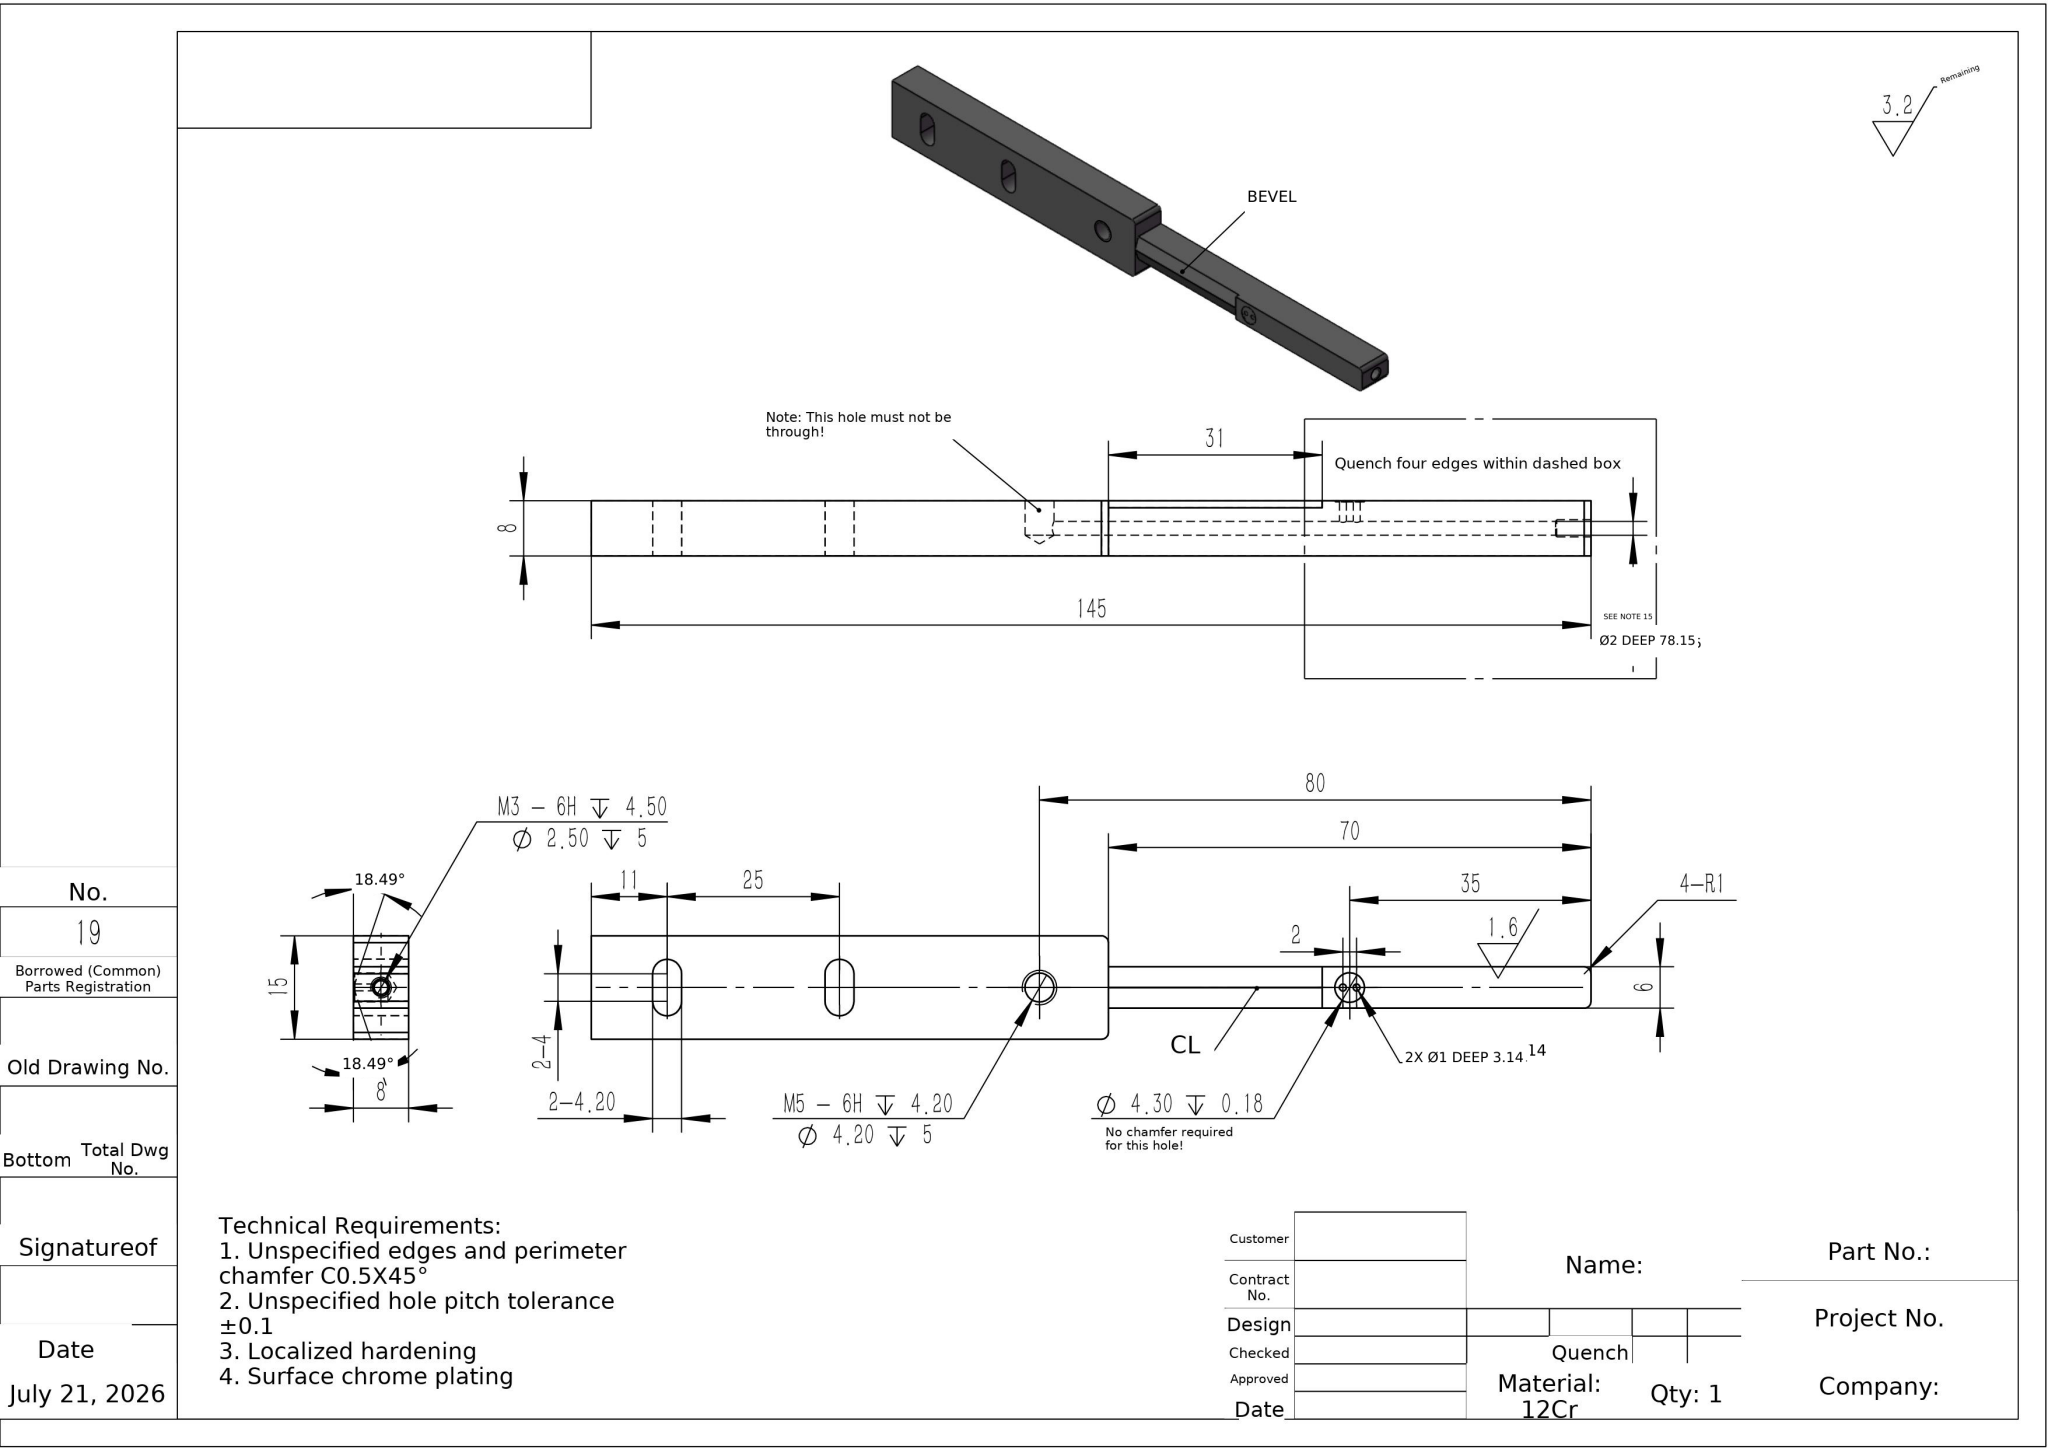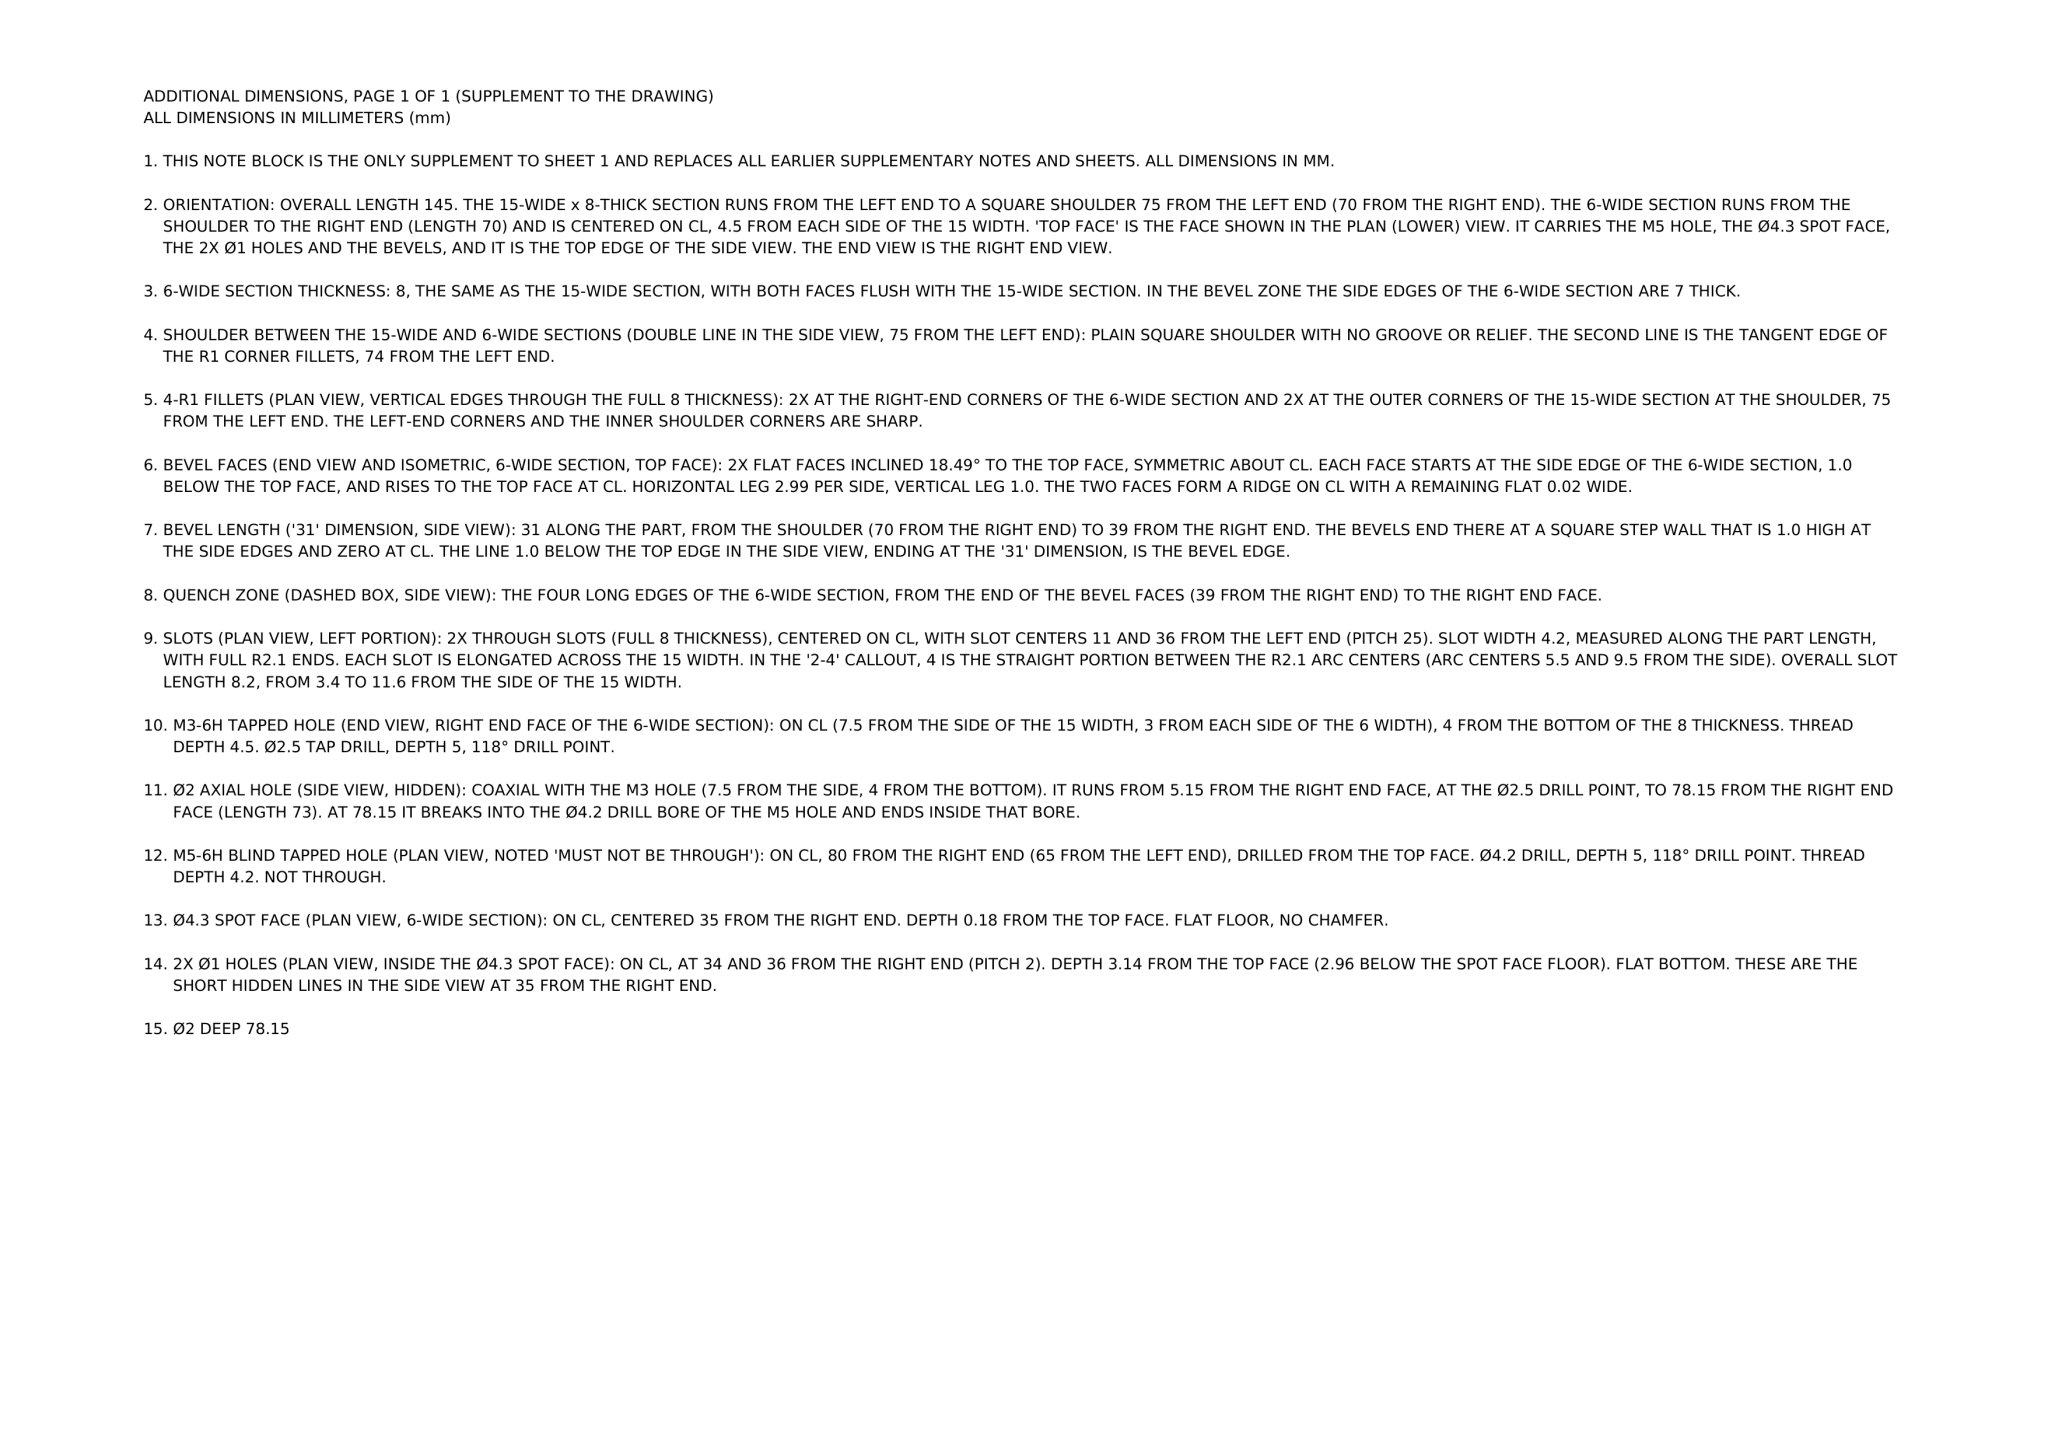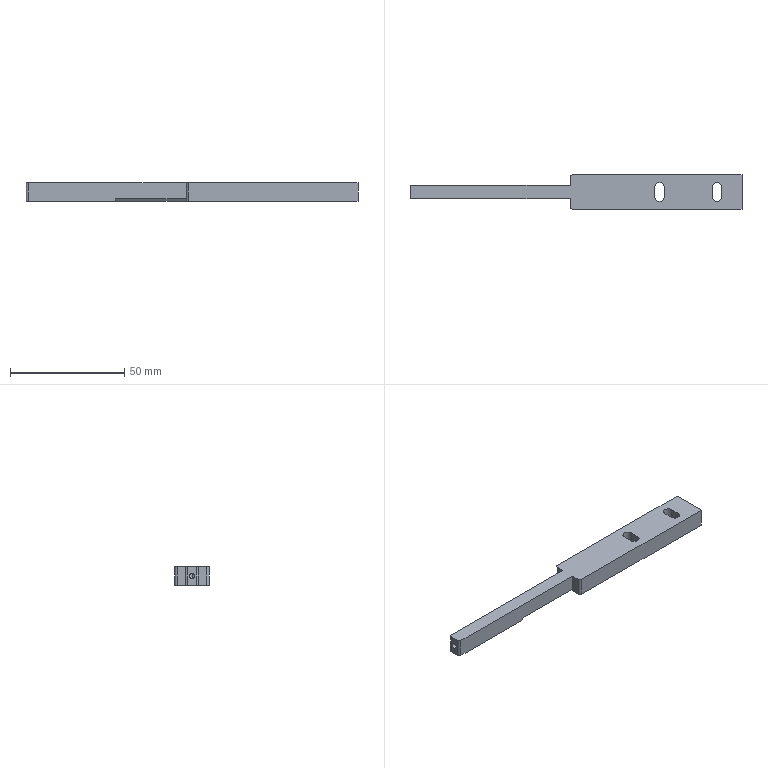Part | NX | mm | 1 solid | 43 faces | box 145 x 15 x 8 mm | volume 11434 mm3 | cylinder 20 | plane 19 | cone 4 | commonest cylinder face diameters 2 x6 4.2 x6 1 x4 2.5 x2 4.3 x2